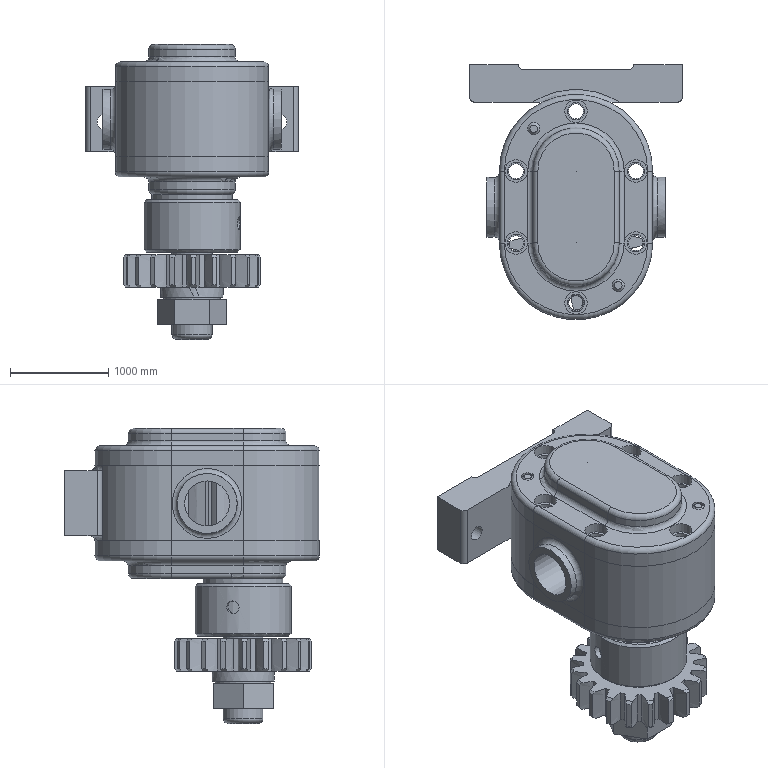Assembly | NX | mm | 13 component files | 31 solids | 471 faces | box 2159 x 2590.8 x 2997.2 mm | volume 4716709751 mm3 | cylinder 184 | plane 130 | other 76 | cone 59 | torus 18 | spline 4 | commonest cylinder face diameters 495.3 x20 1111.25 x20 1397 x20 838.2 x18 101.6 x16 127 x15 177.8 x13 406.4 x12
Bill of materials:
unnamed part 1 | 1 |  | Pinion shaft: a short spur-toothed section with about 9 teeth, a short stepped journal at one end and a long plain cylindrical shaft at the other, with a small elongated slot near the far end of the shaft.
unnamed part 2 | 1 |  | Hexagonal nut-like body with a large central round bore and a thin raised circular collar on one face.
unnamed part 3 | 1 |  | Flat spur gear with about 20 straight teeth and a plain central round bore.
unnamed part 4 | 1 |  | Housing block with an obround outer body and a figure-eight cavity made of two overlapping bores, a ring of holes on the flange face, cylindrical port bosses on two opposite sides, and an attached rectangular mounting bar with holes.
unnamed part 5 | 1 |  | Obround flange plate with a cylindrical stepped boss on one side, two larger bores (one through, one apparently blind with a conical bottom) and eight smaller holes around the edge.
unnamed part 6 | 1 |  | Short gear shaft: a wide toothed section with about 9 teeth and short stepped cylindrical journals at both ends.
unnamed part 7 | 1 |  | Split ring with a rectangular cross-section and a single radial cut through the ring.
unnamed part 8 | 1 |  | Small solid block with an obround (rounded-end) profile and chamfered or rounded edges all around.
unnamed part 9 | 1 |  | Thin-walled plain cylindrical sleeve or tube with a chamfer on one outer end edge.
unnamed part 10 | 1 |  | Obround cover plate with a raised obround pad in the center and eight holes around the flange: six larger holes with counterbores or recesses and two smaller holes.
unnamed part 11 | 2 |  | Solid cylindrical pin with chamfered ends.
unnamed part 12 | 1 |  | Thick-walled cylindrical ring or bushing with chamfered outer edges and two small radial holes through the wall.
Mates:
1. fix | 1 1 component
2. concentric | 10 1 edge | 7youduangai 1 arc
3. concentric | 14 1 edge | 3 1 edge
4. concentric | 7youduangai 1 edge | 6 1 edge
5. concentric | 7youduangai 1 edge | 6 1 edge
6. touch align | 3 1 face | 6 1 face
7. touch align | 2 1 face | 6 1 face
8. concentric | 12 1 edge | 11 1 edge
9. concentric | 13 1 edge | 12 1 edge
10. concentric | 8 1 edge | 7youduangai 1 edge
11. concentric | 4 2 edge | 1 1 edge